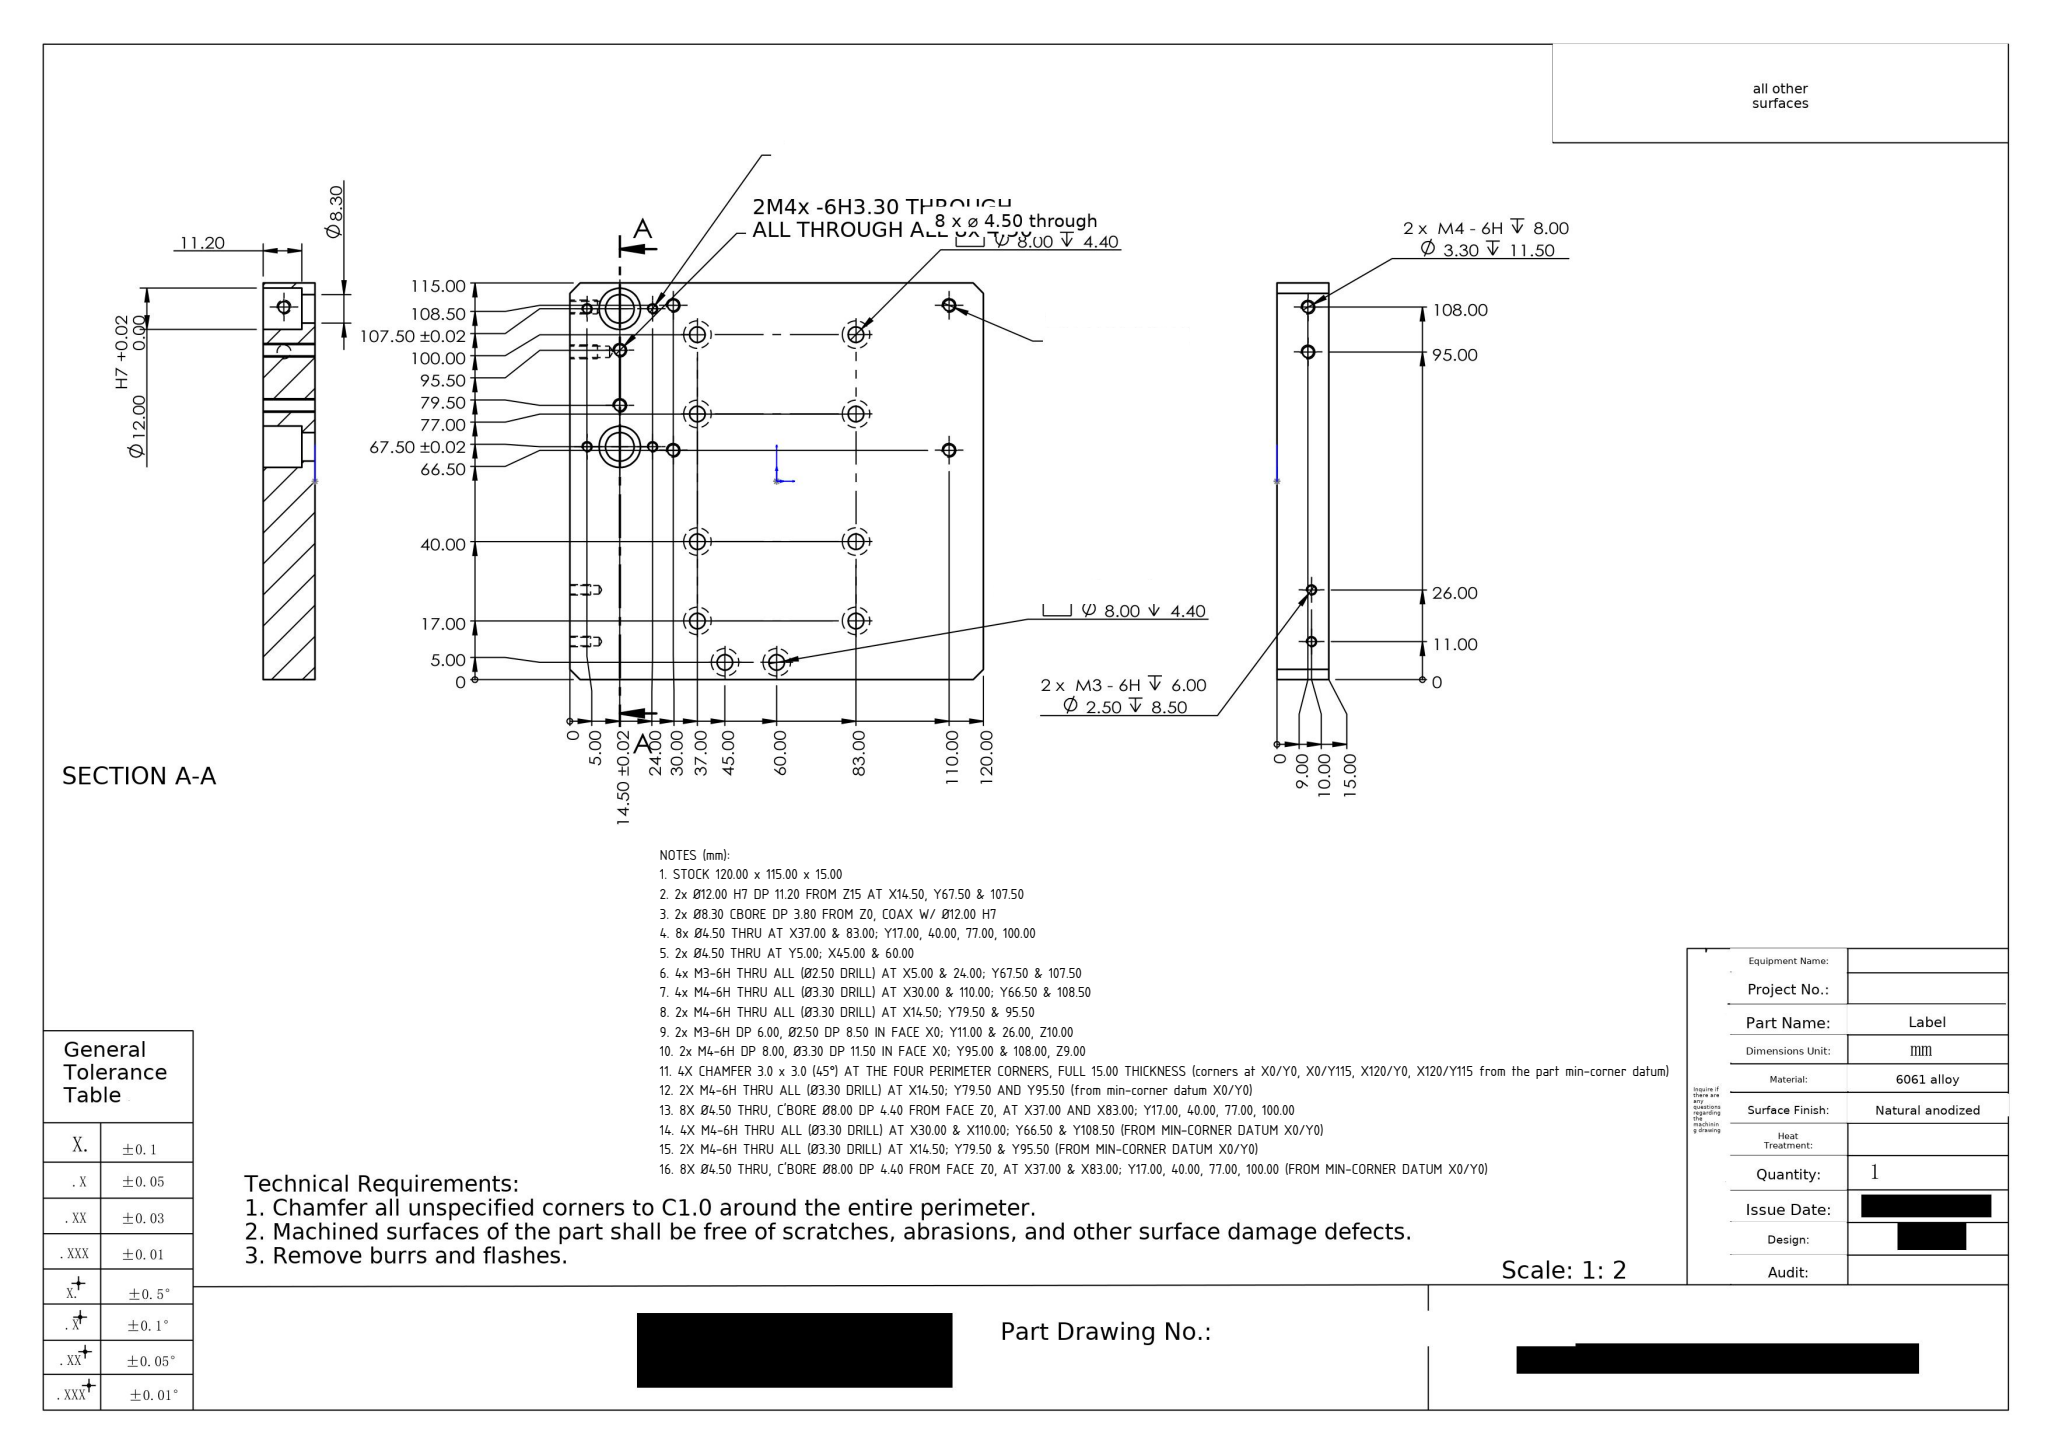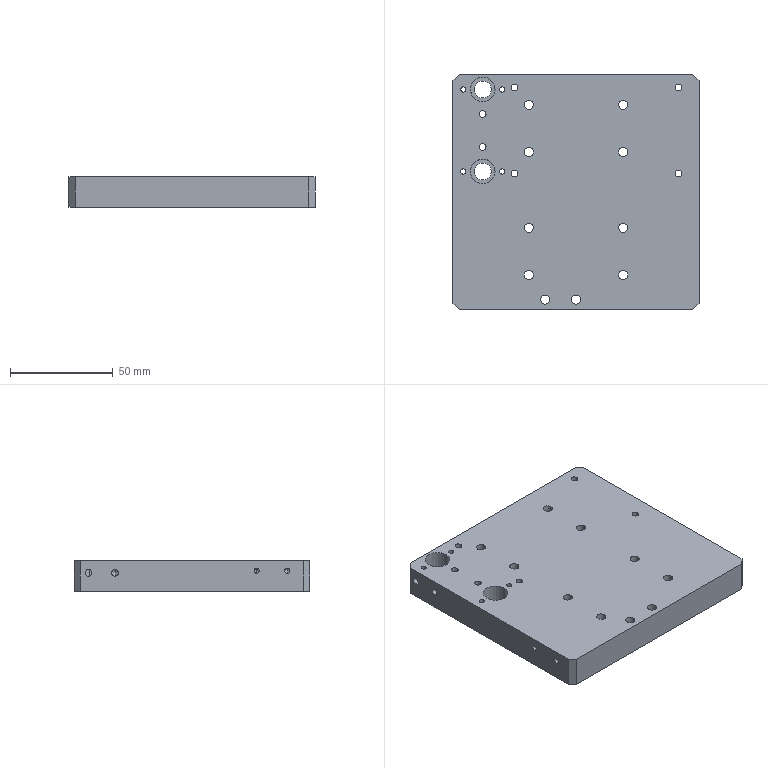Part | SolidWorks | mm | 1 solid | 106 faces | box 120 x 115 x 15 mm | volume 198577 mm3 | cylinder 78 | plane 22 | cone 6 | commonest cylinder face diameters 8 x20 4.5 x20 3.3 x17 2.5 x13 8.3 x4 12 x4
Drawing notes:
STOCK 120.00 x 115.00 x 15.00 | from the solid: bbox_xyz [120,115,15]
2x Ø12.00 H7 DP 11.20 FROM Z15 AT X14.50, Y67.50 & 107.50 | from the solid: Ø12 z-axis cyls L11.2 at (14.5,67.5),(14.5,107.5); planes z=3.8,15
2x Ø8.30 CBORE DP 3.80 FROM Z0, COAX W/ Ø12.00 H7 | from the solid: Ø8.3 z cyls L3.8 at (14.5,67.5),(14.5,107.5); z-plane 3.80
8x Ø4.50 THRU AT X37.00 & 83.00; Y17.00, 40.00, 77.00, 100.00 | from the solid: Ø4.5 z cyls L10.6 at (37/83, 17/40/77/100)
2x Ø4.50 THRU AT Y5.00; X45.00 & 60.00 | from the solid: Ø4.5 z cyls L10.6 at (45,5),(60,5)
4x M3-6H THRU ALL (Ø2.50 DRILL) AT X5.00 & 24.00; Y67.50 & 107.50 | from the solid: Ø2.5 z cyls L15.0 at (5,67.5),(5,107.5),(24,67.5),(24,107.5)
4x M4-6H THRU ALL (Ø3.30 DRILL) AT X30.00 & 110.00; Y66.50 & 108.50 | from the solid: Ø3.3 z cyls L15.0 at (30,66.5),(30,108.5),(110,66.5),(110,108.5)
2x M4-6H THRU ALL (Ø3.30 DRILL) AT X14.50; Y79.50 & 95.50 | from the solid: Ø3.3 z cyls L15.0 at (14.5,79.5),(14.5,95.5)
2x M3-6H DP 6.00, Ø2.50 DP 8.50 IN FACE X0; Y11.00 & 26.00, Z10.00 | from the solid: Ø2.5 x cyls L8.5 at (y11,z10),(y26,z10); cones 118° ref 2.5
2x M4-6H DP 8.00, Ø3.30 DP 11.50 IN FACE X0; Y95.00 & 108.00, Z9.00 | from the solid: Ø3.3 x cyls L11.5 at (y95,z9),(y108,z9); cones 118° ref 3.3
4X CHAMFER 3.0 x 3.0 (45°) AT THE FOUR PERIMETER CORNERS, FULL 15.00 THICKNESS (corners at X0/Y0, X0/Y115, X120/Y0, X120/Y115 from the part min-corner datum) | from the solid: inclined_planes: four 45°/45° faces, size [3.0, 3.0, 15.0], bbox_from [0,0,0], [0,112,0], [117,0,0], [117,112,0]
2X M4-6H THRU ALL (Ø3.30 DRILL) AT X14.50; Y79.50 AND Y95.50 (from min-corner datum X0/Y0) | from the solid: cylinders: hole/bore Ø3.3, axis z at [14.5, 79.5] and [14.5, 95.5], from Z0.0 to Z15.0
8X Ø4.50 THRU, C'BORE Ø8.00 DP 4.40 FROM FACE Z0, AT X37.00 AND X83.00; Y17.00, 40.00, 77.00, 100.00 | from the solid: cylinders: Ø4.5 z-holes from Z4.4 to Z15.0 and Ø8.0 z-bores from Z0.0 to Z4.4 at (37,17),(37,40),(37,77),(37,100),(83,17),(83,40),(83,77),(83,100)
4X M4-6H THRU ALL (Ø3.30 DRILL) AT X30.00 & X110.00; Y66.50 & Y108.50 (FROM MIN-CORNER DATUM X0/Y0) | from the solid: cylinders: hole/bore Ø3.30 axis z at (110,108.5),(110,66.5),(30,108.5),(30,66.5), from z0.0 to z15.0 (full 15.00 thickness)
2X M4-6H THRU ALL (Ø3.30 DRILL) AT X14.50; Y79.50 & Y95.50 (FROM MIN-CORNER DATUM X0/Y0) | from the solid: cylinders: hole/bore Ø3.30 axis z at (14.5,79.5) and (14.5,95.5), from z0.0 to z15.0
8X Ø4.50 THRU, C'BORE Ø8.00 DP 4.40 FROM FACE Z0, AT X37.00 & X83.00; Y17.00, 40.00, 77.00, 100.00 (FROM MIN-CORNER DATUM X0/Y0) | from the solid: cylinders: Ø4.50 axis z from z4.4 to z15.0 and Ø8.00 axis z from z0.0 to z4.4 at (37/83, 17/40/77/100)